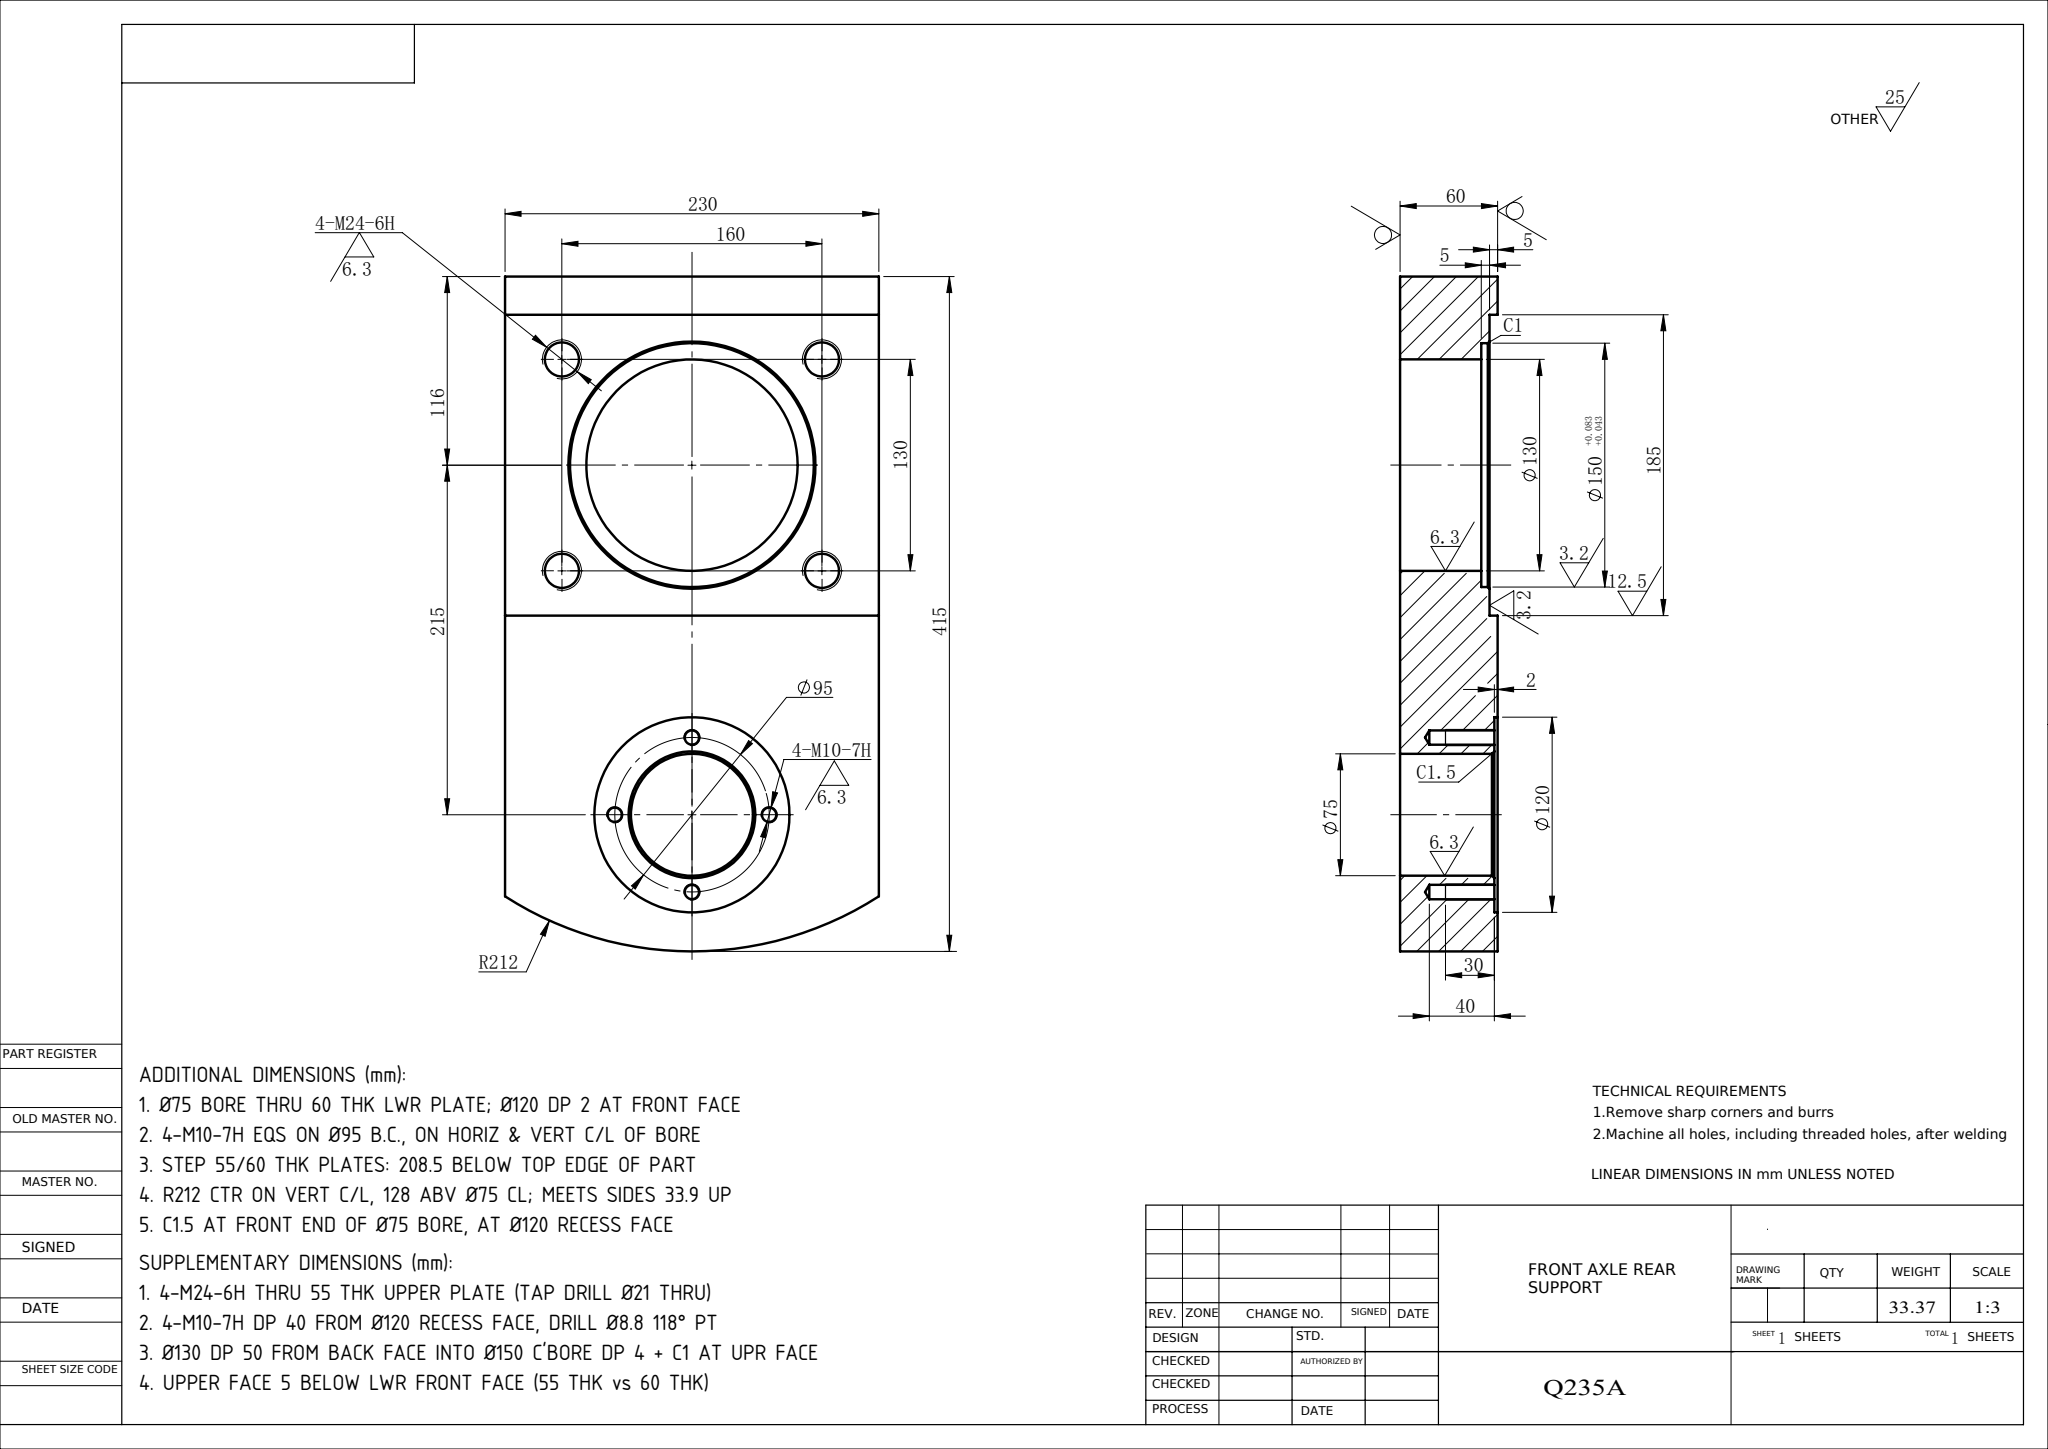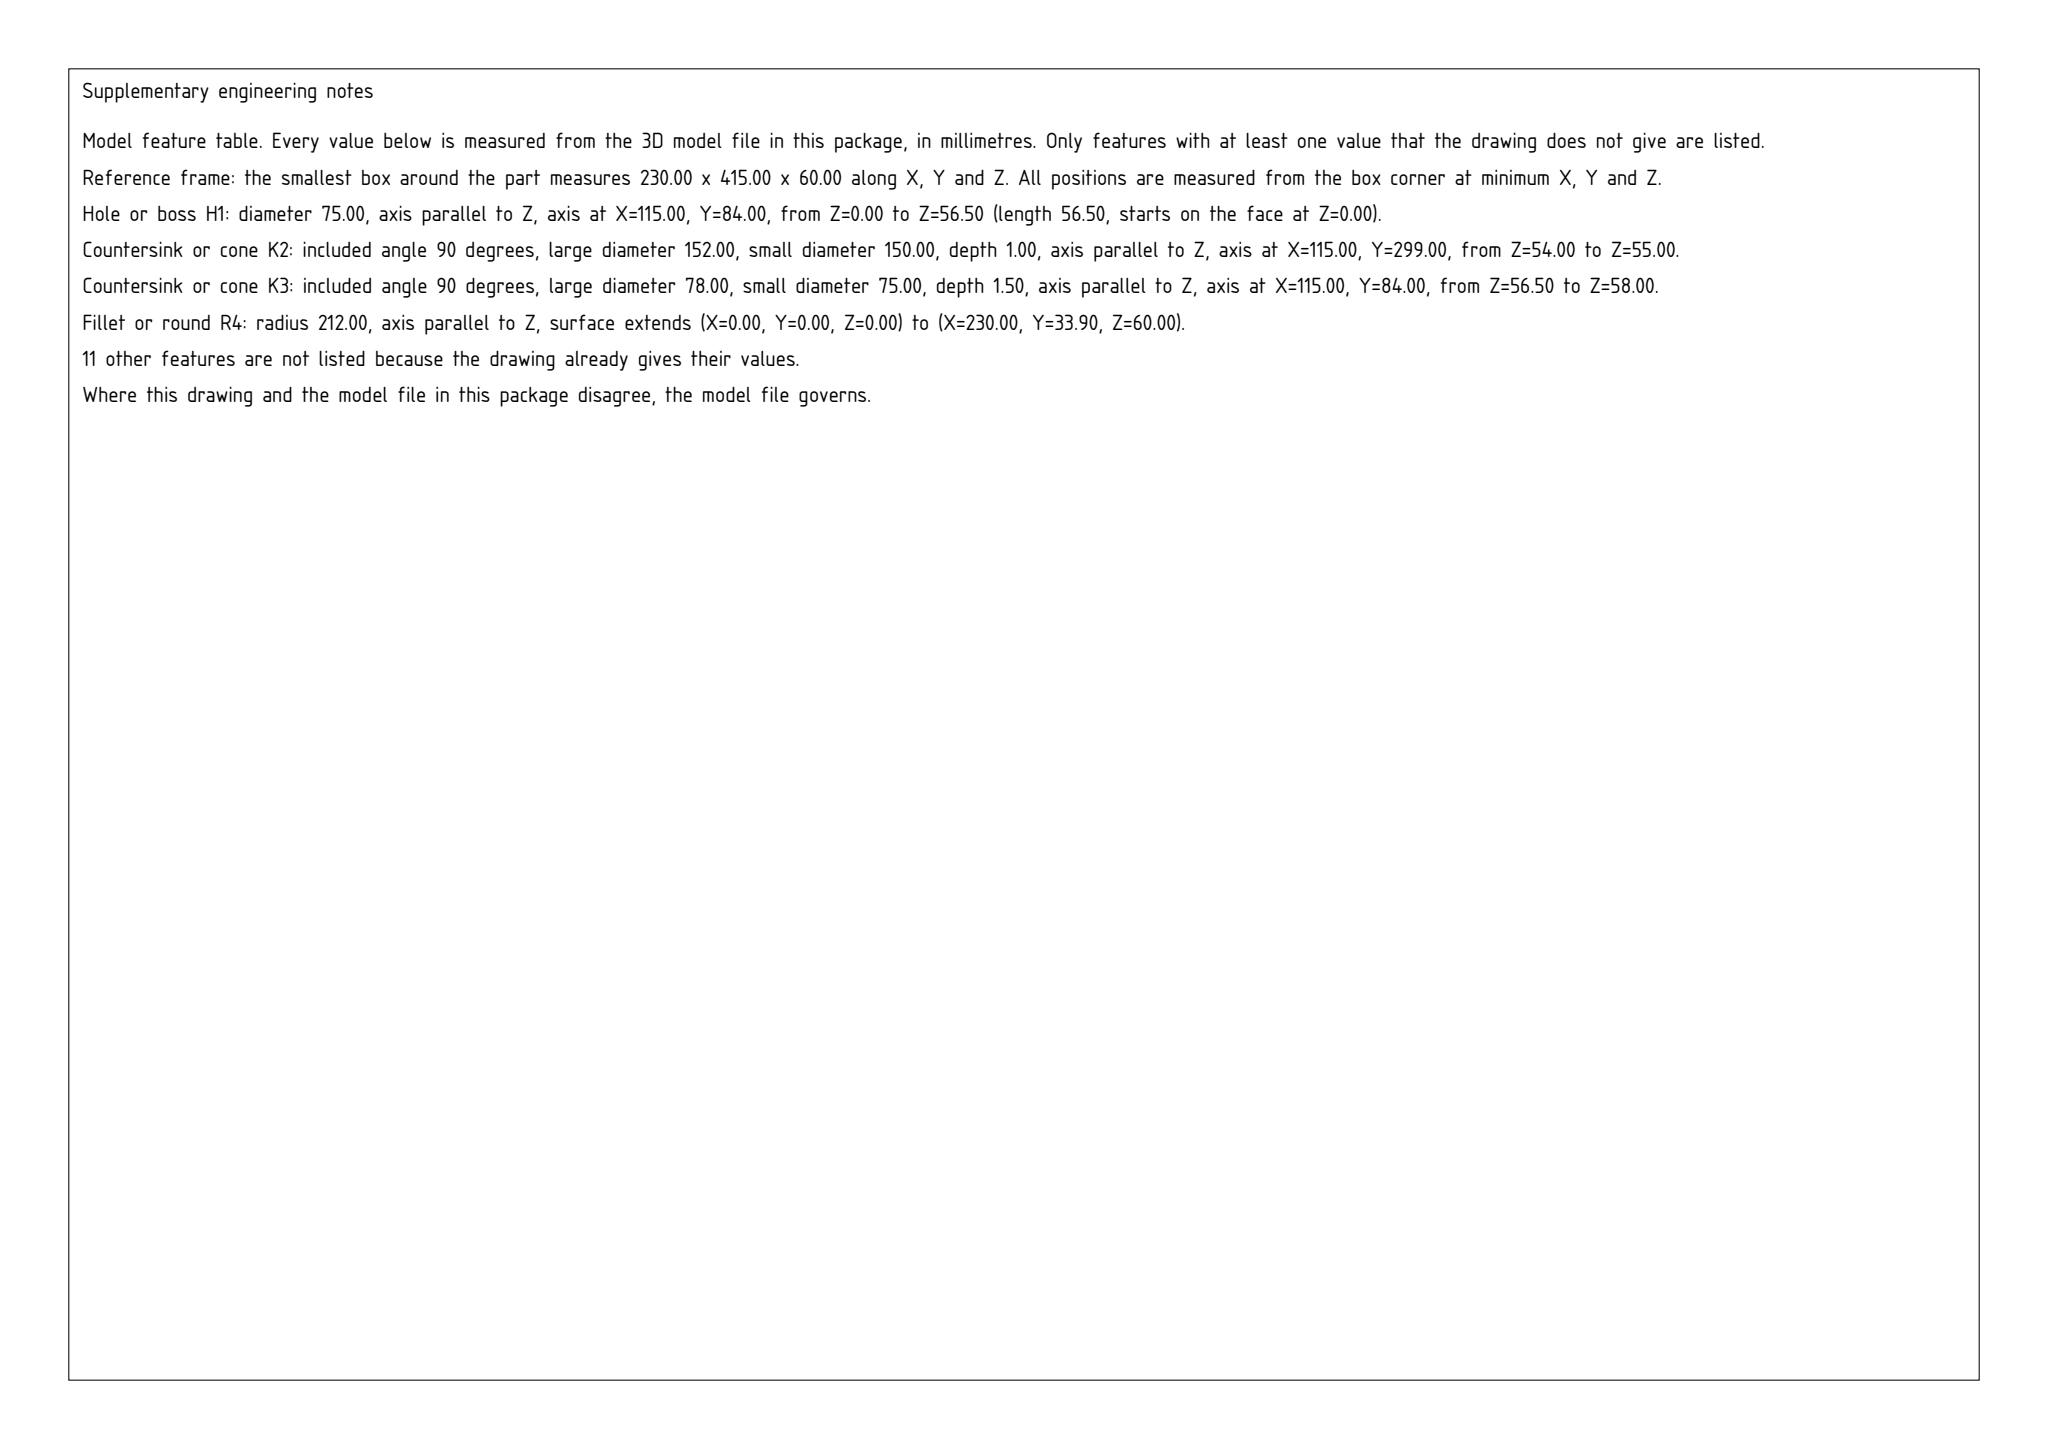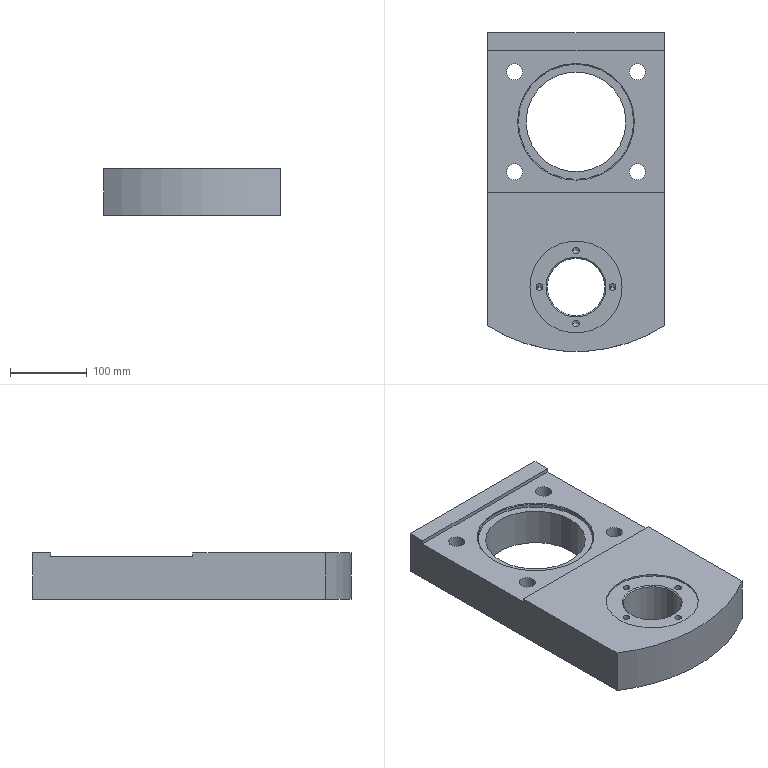Part | SolidWorks | mm | 1 solid | 48 faces | box 230 x 415 x 60 mm | volume 4246133 mm3 | cylinder 25 | cone 12 | plane 11 | commonest cylinder face diameters 8.8 x8 21 x8 120 x2 150 x2 130 x2 75 x2 424 x1
build123d program:
from build123d import *

# Parameters (mm, degrees)
SKETCH2_R           = 37.5
SKETCH2_R_2         = 65
BOSS_EXTRUDE1_DEPTH = 60
SKETCH3_W           = 454.166
SKETCH3_H           = 185
CUT_EXTRUDE1_DEPTH  = 5
SKETCH4_R           = 75
CUT_EXTRUDE2_DEPTH  = 5
CHAMFER1_SIZE       = 1
SKETCH5_R           = 60
CUT_EXTRUDE3_DEPTH  = 2
CHAMFER2_SIZE       = 1.5
M24_TAPPED_HOLE1_D  = 21
CIRPATTERN1_COUNT   = 4


with BuildPart() as part:
    # Sketch2 → Boss-Extrude1 (new body)
    with BuildSketch(Plane.XY):
        with BuildLine():
            Line((-115, 331), (115, 331))
            Line((115, 331), (115, -50.098))
            ThreePointArc((115, -50.098), (0, -84), (-115, -50.098))
            Line((-115, -50.098), (-115, 331))
        make_face()
        Circle(SKETCH2_R, mode=Mode.SUBTRACT)
        with Locations((0, 215)):
            Circle(SKETCH2_R_2, mode=Mode.SUBTRACT)
    extrude(amount=BOSS_EXTRUDE1_DEPTH)

    # Sketch3 → Cut-Extrude1 (cut)
    with BuildSketch(Plane.XY.offset(60)):
        with Locations((-5.485, 215)):
            Rectangle(SKETCH3_W, SKETCH3_H)
    extrude(amount=-CUT_EXTRUDE1_DEPTH, mode=Mode.SUBTRACT)

    # Sketch4 → Cut-Extrude2 (cut)
    with BuildSketch(Plane.XY.offset(55)):
        with Locations((0, 215)):
            Circle(SKETCH4_R)
    extrude(amount=-CUT_EXTRUDE2_DEPTH, mode=Mode.SUBTRACT)

    # Chamfer1
    chamfer1_edges = [part.edges().sort_by_distance(p)[0] for p in [
        (-75, 215, 55),
    ]]
    chamfer(chamfer1_edges, length=CHAMFER1_SIZE)

    # Sketch5 → Cut-Extrude3 (cut)
    with BuildSketch(Plane.XY.offset(60)):
        Circle(SKETCH5_R)
    extrude(amount=-CUT_EXTRUDE3_DEPTH, mode=Mode.SUBTRACT)

    # Chamfer2
    chamfer2_edges = [part.edges().sort_by_distance(p)[0] for p in [
        (-37.5, 0, 58),
    ]]
    chamfer(chamfer2_edges, length=CHAMFER2_SIZE)

    # M24 Tapped Hole1 (through all)
    with Locations(Plane.XY.offset(55)):
        with Locations((-80, 280), (80, 280), (80, 150), (-80, 150)):
            Hole(M24_TAPPED_HOLE1_D / 2)

    # Sketch12 → M10x1.25 Tapped Hole1 (revolve, cut)
    with BuildSketch(Plane(origin=(0, 47.5, 58), x_dir=(0, -1, 0), z_dir=(1, 0, 0))):
        Polygon((0, 0), (0, 42.644), (4.4, 40), (4.4, 0), align=None)
    m10x1_25_tapped_hole1 = revolve(axis=Axis((0, 47.5, 64.35), (0, 0, -1)), mode=Mode.SUBTRACT)

    # CirPattern1: M10x1.25 Tapped Hole1 ×4 about axis
    cirpattern1_axis = Axis((0, 0, 0), (0, 0, 1))
    for i in range(1, CIRPATTERN1_COUNT):
        add(m10x1_25_tapped_hole1.rotate(cirpattern1_axis, i * 360 / CIRPATTERN1_COUNT), mode=Mode.SUBTRACT)


solid = part.part